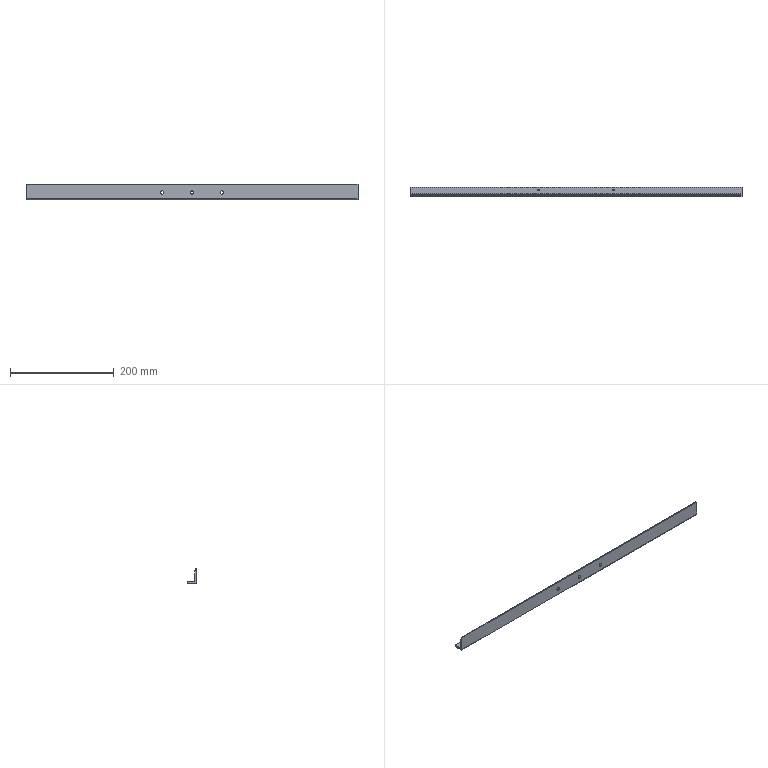Component | SolidWorks | CTM-HVS-52-OA-02-15-1 | 1 solid | 22 faces | box 640 x 18 x 30 mm | volume 105761 mm3 | cylinder 12 | plane 10 | commonest cylinder face diameters 6.6 x6 3.3 x4 4 x2 | material 316L
build123d program:
from build123d import *

# Parameters (mm, degrees)
SKETCH1_W             = 640
SKETCH1_H             = 30
EXTRUDE1_DEPTH        = 2
SKETCH2_W             = 640
SKETCH2_H             = 4
EXTRUDE2_DEPTH        = 14
FILLET1_R             = 2
FILLET2_R             = 2
SKETCH3_R             = 3.3
EXTRUDE3_DEPTH        = 321.657
SKETCH4_W             = 2
SKETCH4_H             = 5
CUT_EXTRUDE1_DEPTH    = 641.376
M4_TAPPED_HOLE1_D     = 3.3
M4_TAPPED_HOLE1_DEPTH = 11.5
M4_TAPPED_HOLE1_TIP   = 0.9914


with BuildPart() as part:
    # Sketch1 → Extrude1 (new, symmetric)
    with BuildSketch(Plane.XY):
        Rectangle(SKETCH1_W, SKETCH1_H)
    extrude(amount=EXTRUDE1_DEPTH, both=True)

    # Sketch2 → Extrude2 (add)
    with BuildSketch(Plane.XY.offset(2)):
        with Locations((0, 13)):
            Rectangle(SKETCH2_W, SKETCH2_H)
    extrude(amount=EXTRUDE2_DEPTH)

    # Fillet1
    fillet1_edges = [part.edges().sort_by_distance(p)[0] for p in [
        (0, 15, -2),
    ]]
    fillet(fillet1_edges, radius=FILLET1_R)

    # Fillet2
    fillet2_edges = [part.edges().sort_by_distance(p)[0] for p in [
        (0, 11, 2),
    ]]
    fillet(fillet2_edges, radius=FILLET2_R)

    # Sketch3 → Extrude3 (cut, through all)
    with BuildSketch(Plane.XY.offset(2)):
        with Locations((-57.5, 1)):
            Circle(SKETCH3_R)
        with Locations((0, 1)):
            Circle(SKETCH3_R)
    extrude3 = extrude(amount=-EXTRUDE3_DEPTH, mode=Mode.SUBTRACT)

    # Mirror1: Extrude3 across plane
    add(extrude3.mirror(Plane(origin=(0, 0, 0), x_dir=(0, 0, 1), z_dir=(1, 0, 0))), mode=Mode.SUBTRACT)

    # Sketch4 → Cut-Extrude1 (cut, through all)
    with BuildSketch(Plane.ZY.offset(320)):
        with Locations((1, -12.5)):
            Rectangle(SKETCH4_W, SKETCH4_H)
    extrude(amount=-CUT_EXTRUDE1_DEPTH, mode=Mode.SUBTRACT)

    # M4 Tapped Hole1
    with Locations(Plane.XZ.offset(-11)):
        with Locations((-72.5, 11), (72.5, 11)):
            Hole(M4_TAPPED_HOLE1_D / 2, depth=M4_TAPPED_HOLE1_DEPTH)
            with Locations((0, 0, -(M4_TAPPED_HOLE1_DEPTH + M4_TAPPED_HOLE1_TIP / 2))):  # 118° drill point
                Cone(0, M4_TAPPED_HOLE1_D / 2, M4_TAPPED_HOLE1_TIP, mode=Mode.SUBTRACT)


solid = part.part

# Placed as in the assembly
solid = solid.moved(Location((-22.307, -58.557, 37.5), (-90, 0, 0)))
STEP:
#1=CARTESIAN_POINT('',(-3.733,-1.807,0.8858));
#2=VERTEX_POINT('',#1);
#3=CARTESIAN_POINT('',(-3.733,-1.937,0.8858));
#4=VERTEX_POINT('',#3);
#5=CARTESIAN_POINT('',(-3.733,-1.872,0.8858));
#6=DIRECTION('',(-0.,-0.,1.));
#7=DIRECTION('',(0.,-1.,0.));
#8=AXIS2_PLACEMENT_3D('',#5,#6,#7);
#9=CIRCLE('',#8,0.06496);
#10=EDGE_CURVE('',#2,#4,#9,.T.);
#11=ORIENTED_EDGE('',*,*,#10,.F.);
#12=CARTESIAN_POINT('',(-3.733,-1.807,1.043));
#13=VERTEX_POINT('',#12);
#14=CARTESIAN_POINT('',(-3.733,-1.807,1.043));
#15=DIRECTION('',(-0.,-0.,1.));
#16=VECTOR('',#15,39.37);
#17=LINE('',#14,#16);
#18=EDGE_CURVE('',#2,#13,#17,.T.);
#19=ORIENTED_EDGE('',*,*,#18,.T.);
#20=CARTESIAN_POINT('',(-3.733,-1.937,1.043));
#21=VERTEX_POINT('',#20);
#22=CARTESIAN_POINT('',(-3.733,-1.872,1.043));
#23=DIRECTION('',(-0.,-0.,1.));
#24=DIRECTION('',(0.,-1.,0.));
#25=AXIS2_PLACEMENT_3D('',#22,#23,#24);
#26=CIRCLE('',#25,0.06496);
#27=EDGE_CURVE('',#13,#21,#26,.T.);
#28=ORIENTED_EDGE('',*,*,#27,.T.);
#29=CARTESIAN_POINT('',(-3.733,-1.937,1.043));
#30=DIRECTION('',(-0.,-0.,1.));
#31=VECTOR('',#30,39.37);
#32=LINE('',#29,#31);
#33=EDGE_CURVE('',#4,#21,#32,.T.);
#34=ORIENTED_EDGE('',*,*,#33,.F.);
#35=EDGE_LOOP('',(#11,#19,#28,#34));
#36=FACE_OUTER_BOUND('',#35,.T.);
#37=CARTESIAN_POINT('',(-3.733,-1.872,1.043));
#38=DIRECTION('',(-0.,-0.,1.));
#39=DIRECTION('',(0.,-1.,0.));
#40=AXIS2_PLACEMENT_3D('',#37,#38,#39);
#41=CYLINDRICAL_SURFACE('',#40,0.06496);
#42=ADVANCED_FACE('',(#36),#41,.F.);
#43=CARTESIAN_POINT('',(1.976,-1.807,0.8858));
#44=VERTEX_POINT('',#43);
#45=CARTESIAN_POINT('',(1.976,-1.937,0.8858));
#46=VERTEX_POINT('',#45);
#47=CARTESIAN_POINT('',(1.976,-1.872,0.8858));
#48=DIRECTION('',(-0.,-0.,1.));
#49=DIRECTION('',(0.,-1.,0.));
#50=AXIS2_PLACEMENT_3D('',#47,#48,#49);
#51=CIRCLE('',#50,0.06496);
#52=EDGE_CURVE('',#44,#46,#51,.T.);
#53=ORIENTED_EDGE('',*,*,#52,.F.);
#54=CARTESIAN_POINT('',(1.976,-1.807,1.043));
#55=VERTEX_POINT('',#54);
#56=CARTESIAN_POINT('',(1.976,-1.807,1.043));
#57=DIRECTION('',(-0.,-0.,1.));
#58=VECTOR('',#57,39.37);
#59=LINE('',#56,#58);
#60=EDGE_CURVE('',#44,#55,#59,.T.);
#61=ORIENTED_EDGE('',*,*,#60,.T.);
#62=CARTESIAN_POINT('',(1.976,-1.937,1.043));
#63=VERTEX_POINT('',#62);
#64=CARTESIAN_POINT('',(1.976,-1.872,1.043));
#65=DIRECTION('',(-0.,-0.,1.));
#66=DIRECTION('',(0.,-1.,0.));
#67=AXIS2_PLACEMENT_3D('',#64,#65,#66);
#68=CIRCLE('',#67,0.06496);
#69=EDGE_CURVE('',#55,#63,#68,.T.);
#70=ORIENTED_EDGE('',*,*,#69,.T.);
#71=CARTESIAN_POINT('',(1.976,-1.937,1.043));
#72=DIRECTION('',(-0.,-0.,1.));
#73=VECTOR('',#72,39.37);
#74=LINE('',#71,#73);
#75=EDGE_CURVE('',#46,#63,#74,.T.);
#76=ORIENTED_EDGE('',*,*,#75,.F.);
#77=EDGE_LOOP('',(#53,#61,#70,#76));
#78=FACE_OUTER_BOUND('',#77,.T.);
#79=CARTESIAN_POINT('',(1.976,-1.872,1.043));
#80=DIRECTION('',(-0.,-0.,1.));
#81=DIRECTION('',(0.,-1.,0.));
#82=AXIS2_PLACEMENT_3D('',#79,#80,#81);
#83=CYLINDRICAL_SURFACE('',#82,0.06496);
#84=ADVANCED_FACE('',(#78),#83,.F.);
#85=CARTESIAN_POINT('',(1.515,-2.384,1.437));
#86=VERTEX_POINT('',#85);
#87=CARTESIAN_POINT('',(1.256,-2.384,1.437));
#88=VERTEX_POINT('',#87);
#89=CARTESIAN_POINT('',(1.386,-2.384,1.437));
#90=DIRECTION('',(-0.,-1.,-0.));
#91=DIRECTION('',(-1.,0.,-0.));
#92=AXIS2_PLACEMENT_3D('',#89,#90,#91);
#93=CIRCLE('',#92,0.1299);
#94=EDGE_CURVE('',#86,#88,#93,.T.);
#95=ORIENTED_EDGE('',*,*,#94,.T.);
#96=CARTESIAN_POINT('',(1.256,-2.227,1.437));
#97=VERTEX_POINT('',#96);
#98=CARTESIAN_POINT('',(1.256,-2.384,1.437));
#99=DIRECTION('',(0.,1.,0.));
#100=VECTOR('',#99,39.37);
#101=LINE('',#98,#100);
#102=EDGE_CURVE('',#88,#97,#101,.T.);
#103=ORIENTED_EDGE('',*,*,#102,.T.);
#104=CARTESIAN_POINT('',(1.515,-2.227,1.437));
#105=VERTEX_POINT('',#104);
#106=CARTESIAN_POINT('',(1.386,-2.227,1.437));
#107=DIRECTION('',(-0.,-1.,-0.));
#108=DIRECTION('',(-1.,0.,-0.));
#109=AXIS2_PLACEMENT_3D('',#106,#107,#108);
#110=CIRCLE('',#109,0.1299);
#111=EDGE_CURVE('',#105,#97,#110,.T.);
#112=ORIENTED_EDGE('',*,*,#111,.F.);
#113=CARTESIAN_POINT('',(1.515,-2.384,1.437));
#114=DIRECTION('',(0.,1.,0.));
#115=VECTOR('',#114,39.37);
#116=LINE('',#113,#115);
#117=EDGE_CURVE('',#86,#105,#116,.T.);
#118=ORIENTED_EDGE('',*,*,#117,.F.);
#119=EDGE_LOOP('',(#95,#103,#112,#118));
#120=FACE_OUTER_BOUND('',#119,.T.);
#121=CARTESIAN_POINT('',(1.386,-2.384,1.437));
#122=DIRECTION('',(0.,1.,0.));
#123=DIRECTION('',(1.,0.,0.));
#124=AXIS2_PLACEMENT_3D('',#121,#122,#123);
#125=CYLINDRICAL_SURFACE('',#124,0.1299);
#126=ADVANCED_FACE('',(#120),#125,.F.);
#127=CARTESIAN_POINT('',(-1.008,-2.384,1.437));
#128=VERTEX_POINT('',#127);
#129=CARTESIAN_POINT('',(-0.7483,-2.384,1.437));
#130=VERTEX_POINT('',#129);
#131=CARTESIAN_POINT('',(-0.8782,-2.384,1.437));
#132=DIRECTION('',(0.,1.,0.));
#133=DIRECTION('',(1.,0.,0.));
#134=AXIS2_PLACEMENT_3D('',#131,#132,#133);
#135=CIRCLE('',#134,0.1299);
#136=EDGE_CURVE('',#128,#130,#135,.T.);
#137=ORIENTED_EDGE('',*,*,#136,.F.);
#138=CARTESIAN_POINT('',(-1.008,-2.227,1.437));
#139=VERTEX_POINT('',#138);
#140=CARTESIAN_POINT('',(-1.008,-2.384,1.437));
#141=DIRECTION('',(0.,1.,0.));
#142=VECTOR('',#141,39.37);
#143=LINE('',#140,#142);
#144=EDGE_CURVE('',#128,#139,#143,.T.);
#145=ORIENTED_EDGE('',*,*,#144,.T.);
#146=CARTESIAN_POINT('',(-0.7483,-2.227,1.437));
#147=VERTEX_POINT('',#146);
#148=CARTESIAN_POINT('',(-0.8782,-2.227,1.437));
#149=DIRECTION('',(0.,1.,0.));
#150=DIRECTION('',(1.,0.,0.));
#151=AXIS2_PLACEMENT_3D('',#148,#149,#150);
#152=CIRCLE('',#151,0.1299);
#153=EDGE_CURVE('',#139,#147,#152,.T.);
#154=ORIENTED_EDGE('',*,*,#153,.T.);
#155=CARTESIAN_POINT('',(-0.7483,-2.384,1.437));
#156=DIRECTION('',(0.,1.,0.));
#157=VECTOR('',#156,39.37);
#158=LINE('',#155,#157);
#159=EDGE_CURVE('',#130,#147,#158,.T.);
#160=ORIENTED_EDGE('',*,*,#159,.F.);
#161=EDGE_LOOP('',(#137,#145,#154,#160));
#162=FACE_OUTER_BOUND('',#161,.T.);
#163=CARTESIAN_POINT('',(-0.8782,-2.384,1.437));
#164=DIRECTION('',(0.,1.,0.));
#165=DIRECTION('',(1.,0.,0.));
#166=AXIS2_PLACEMENT_3D('',#163,#164,#165);
#167=CYLINDRICAL_SURFACE('',#166,0.1299);
#168=ADVANCED_FACE('',(#162),#167,.F.);
#169=CARTESIAN_POINT('',(-3.272,-2.384,1.437));
#170=VERTEX_POINT('',#169);
#171=CARTESIAN_POINT('',(-3.012,-2.384,1.437));
#172=VERTEX_POINT('',#171);
#173=CARTESIAN_POINT('',(-3.142,-2.384,1.437));
#174=DIRECTION('',(0.,1.,0.));
#175=DIRECTION('',(1.,0.,0.));
#176=AXIS2_PLACEMENT_3D('',#173,#174,#175);
#177=CIRCLE('',#176,0.1299);
#178=EDGE_CURVE('',#170,#172,#177,.T.);
#179=ORIENTED_EDGE('',*,*,#178,.F.);
#180=CARTESIAN_POINT('',(-3.272,-2.227,1.437));
#181=VERTEX_POINT('',#180);
#182=CARTESIAN_POINT('',(-3.272,-2.384,1.437));
#183=DIRECTION('',(0.,1.,0.));
#184=VECTOR('',#183,39.37);
#185=LINE('',#182,#184);
#186=EDGE_CURVE('',#170,#181,#185,.T.);
#187=ORIENTED_EDGE('',*,*,#186,.T.);
#188=CARTESIAN_POINT('',(-3.012,-2.227,1.437));
#189=VERTEX_POINT('',#188);
#190=CARTESIAN_POINT('',(-3.142,-2.227,1.437));
#191=DIRECTION('',(0.,1.,0.));
#192=DIRECTION('',(1.,0.,0.));
#193=AXIS2_PLACEMENT_3D('',#190,#191,#192);
#194=CIRCLE('',#193,0.1299);
#195=EDGE_CURVE('',#181,#189,#194,.T.);
#196=ORIENTED_EDGE('',*,*,#195,.T.);
#197=CARTESIAN_POINT('',(-3.012,-2.384,1.437));
#198=DIRECTION('',(0.,1.,0.));
#199=VECTOR('',#198,39.37);
#200=LINE('',#197,#199);
#201=EDGE_CURVE('',#172,#189,#200,.T.);
#202=ORIENTED_EDGE('',*,*,#201,.F.);
#203=EDGE_LOOP('',(#179,#187,#196,#202));
#204=FACE_OUTER_BOUND('',#203,.T.);
#205=CARTESIAN_POINT('',(-3.142,-2.384,1.437));
#206=DIRECTION('',(0.,1.,0.));
#207=DIRECTION('',(1.,0.,0.));
#208=AXIS2_PLACEMENT_3D('',#205,#206,#207);
#209=CYLINDRICAL_SURFACE('',#208,0.1299);
#210=ADVANCED_FACE('',(#204),#209,.F.);
#211=CARTESIAN_POINT('',(-13.477,-1.675,1.043));
#212=VERTEX_POINT('',#211);
#213=CARTESIAN_POINT('',(-13.477,-2.148,1.043));
#214=VERTEX_POINT('',#213);
#215=CARTESIAN_POINT('',(-13.477,-1.675,1.043));
#216=DIRECTION('',(-0.,-1.,-0.));
#217=VECTOR('',#216,39.37);
#218=LINE('',#215,#217);
#219=EDGE_CURVE('',#212,#214,#218,.T.);
#220=ORIENTED_EDGE('',*,*,#219,.T.);
#221=CARTESIAN_POINT('',(11.72,-2.148,1.043));
#222=VERTEX_POINT('',#221);
#223=CARTESIAN_POINT('',(-13.477,-2.148,1.043));
#224=DIRECTION('',(1.,-0.,0.));
#225=VECTOR('',#224,39.37);
#226=LINE('',#223,#225);
#227=EDGE_CURVE('',#214,#222,#226,.T.);
#228=ORIENTED_EDGE('',*,*,#227,.T.);
#229=CARTESIAN_POINT('',(11.72,-1.675,1.043));
#230=VERTEX_POINT('',#229);
#231=CARTESIAN_POINT('',(11.72,-1.675,1.043));
#232=DIRECTION('',(-0.,-1.,-0.));
#233=VECTOR('',#232,39.37);
#234=LINE('',#231,#233);
#235=EDGE_CURVE('',#230,#222,#234,.T.);
#236=ORIENTED_EDGE('',*,*,#235,.F.);
#237=CARTESIAN_POINT('',(-13.477,-1.675,1.043));
#238=DIRECTION('',(1.,-0.,0.));
#239=VECTOR('',#238,39.37);
#240=LINE('',#237,#239);
#241=EDGE_CURVE('',#212,#230,#240,.T.);
#242=ORIENTED_EDGE('',*,*,#241,.F.);
#243=EDGE_LOOP('',(#220,#228,#236,#242));
#244=FACE_OUTER_BOUND('',#243,.T.);
#245=CARTESIAN_POINT('',(1.976,-1.872,1.043));
#246=DIRECTION('',(-0.,-0.,1.));
#247=DIRECTION('',(0.,-1.,0.));
#248=AXIS2_PLACEMENT_3D('',#245,#246,#247);
#249=CIRCLE('',#248,0.06496);
#250=EDGE_CURVE('',#63,#55,#249,.T.);
#251=ORIENTED_EDGE('',*,*,#250,.F.);
#252=ORIENTED_EDGE('',*,*,#69,.F.);
#253=EDGE_LOOP('',(#251,#252));
#254=FACE_BOUND('',#253,.T.);
#255=CARTESIAN_POINT('',(-3.733,-1.872,1.043));
#256=DIRECTION('',(-0.,-0.,1.));
#257=DIRECTION('',(0.,-1.,0.));
#258=AXIS2_PLACEMENT_3D('',#255,#256,#257);
#259=CIRCLE('',#258,0.06496);
#260=EDGE_CURVE('',#21,#13,#259,.T.);
#261=ORIENTED_EDGE('',*,*,#260,.F.);
#262=ORIENTED_EDGE('',*,*,#27,.F.);
#263=EDGE_LOOP('',(#261,#262));
#264=FACE_BOUND('',#263,.T.);
#265=CARTESIAN_POINT('',(-13.477,-1.675,1.043));
#266=DIRECTION('',(0.,0.,-1.));
#267=DIRECTION('',(0.,1.,0.));
#268=AXIS2_PLACEMENT_3D('',#265,#266,#267);
#269=PLANE('',#268);
#270=ADVANCED_FACE('',(#244,#254,#264),#269,.F.);
#271=CARTESIAN_POINT('',(11.72,-2.227,1.87));
#272=VERTEX_POINT('',#271);
#273=CARTESIAN_POINT('',(-13.477,-2.227,1.87));
#274=VERTEX_POINT('',#273);
#275=CARTESIAN_POINT('',(11.72,-2.227,1.87));
#276=DIRECTION('',(-1.,0.,-0.));
#277=VECTOR('',#276,39.37);
#278=LINE('',#275,#277);
#279=EDGE_CURVE('',#272,#274,#278,.T.);
#280=ORIENTED_EDGE('',*,*,#279,.F.);
#281=CARTESIAN_POINT('',(11.72,-2.227,1.122));
#282=VERTEX_POINT('',#281);
#283=CARTESIAN_POINT('',(11.72,-2.227,0.8858));
#284=DIRECTION('',(0.,0.,-1.));
#285=VECTOR('',#284,39.37);
#286=LINE('',#283,#285);
#287=EDGE_CURVE('',#272,#282,#286,.T.);
#288=ORIENTED_EDGE('',*,*,#287,.T.);
#289=CARTESIAN_POINT('',(-13.477,-2.227,1.122));
#290=VERTEX_POINT('',#289);
#291=CARTESIAN_POINT('',(11.72,-2.227,1.122));
#292=DIRECTION('',(-1.,0.,-0.));
#293=VECTOR('',#292,39.37);
#294=LINE('',#291,#293);
#295=EDGE_CURVE('',#282,#290,#294,.T.);
#296=ORIENTED_EDGE('',*,*,#295,.T.);
#297=CARTESIAN_POINT('',(-13.477,-2.227,0.8858));
#298=DIRECTION('',(-0.,-0.,1.));
#299=VECTOR('',#298,39.37);
#300=LINE('',#297,#299);
#301=EDGE_CURVE('',#290,#274,#300,.T.);
#302=ORIENTED_EDGE('',*,*,#301,.T.);
#303=EDGE_LOOP('',(#280,#288,#296,#302));
#304=FACE_OUTER_BOUND('',#303,.T.);
#305=CARTESIAN_POINT('',(-3.142,-2.227,1.437));
#306=DIRECTION('',(0.,1.,0.));
#307=DIRECTION('',(1.,0.,0.));
#308=AXIS2_PLACEMENT_3D('',#305,#306,#307);
#309=CIRCLE('',#308,0.1299);
#310=EDGE_CURVE('',#189,#181,#309,.T.);
#311=ORIENTED_EDGE('',*,*,#310,.F.);
#312=ORIENTED_EDGE('',*,*,#195,.F.);
#313=EDGE_LOOP('',(#311,#312));
#314=FACE_BOUND('',#313,.T.);
#315=CARTESIAN_POINT('',(-0.8782,-2.227,1.437));
#316=DIRECTION('',(0.,1.,0.));
#317=DIRECTION('',(1.,0.,0.));
#318=AXIS2_PLACEMENT_3D('',#315,#316,#317);
#319=CIRCLE('',#318,0.1299);
#320=EDGE_CURVE('',#147,#139,#319,.T.);
#321=ORIENTED_EDGE('',*,*,#320,.F.);
#322=ORIENTED_EDGE('',*,*,#153,.F.);
#323=EDGE_LOOP('',(#321,#322));
#324=FACE_BOUND('',#323,.T.);
#325=ORIENTED_EDGE('',*,*,#111,.T.);
#326=CARTESIAN_POINT('',(1.386,-2.227,1.437));
#327=DIRECTION('',(-0.,-1.,-0.));
#328=DIRECTION('',(-1.,0.,-0.));
#329=AXIS2_PLACEMENT_3D('',#326,#327,#328);
#330=CIRCLE('',#329,0.1299);
#331=EDGE_CURVE('',#97,#105,#330,.T.);
#332=ORIENTED_EDGE('',*,*,#331,.T.);
#333=EDGE_LOOP('',(#325,#332));
#334=FACE_BOUND('',#333,.T.);
#335=CARTESIAN_POINT('',(11.72,-2.227,2.067));
#336=DIRECTION('',(0.,1.,0.));
#337=DIRECTION('',(1.,-0.,0.));
#338=AXIS2_PLACEMENT_3D('',#335,#336,#337);
#339=PLANE('',#338);
#340=ADVANCED_FACE('',(#304,#314,#324,#334),#339,.T.);
#341=CARTESIAN_POINT('',(-13.477,-2.384,0.9646));
#342=VERTEX_POINT('',#341);
#343=CARTESIAN_POINT('',(-13.477,-2.384,2.067));
#344=VERTEX_POINT('',#343);
#345=CARTESIAN_POINT('',(-13.477,-2.384,0.8858));
#346=DIRECTION('',(-0.,-0.,1.));
#347=VECTOR('',#346,39.37);
#348=LINE('',#345,#347);
#349=EDGE_CURVE('',#342,#344,#348,.T.);
#350=ORIENTED_EDGE('',*,*,#349,.F.);
#351=CARTESIAN_POINT('',(11.72,-2.384,0.9646));
#352=VERTEX_POINT('',#351);
#353=CARTESIAN_POINT('',(11.72,-2.384,0.9646));
#354=DIRECTION('',(1.,-0.,0.));
#355=VECTOR('',#354,39.37);
#356=LINE('',#353,#355);
#357=EDGE_CURVE('',#342,#352,#356,.T.);
#358=ORIENTED_EDGE('',*,*,#357,.T.);
#359=CARTESIAN_POINT('',(11.72,-2.384,2.067));
#360=VERTEX_POINT('',#359);
#361=CARTESIAN_POINT('',(11.72,-2.384,0.8858));
#362=DIRECTION('',(0.,0.,-1.));
#363=VECTOR('',#362,39.37);
#364=LINE('',#361,#363);
#365=EDGE_CURVE('',#360,#352,#364,.T.);
#366=ORIENTED_EDGE('',*,*,#365,.F.);
#367=CARTESIAN_POINT('',(-13.477,-2.384,2.067));
#368=DIRECTION('',(1.,-0.,0.));
#369=VECTOR('',#368,39.37);
#370=LINE('',#367,#369);
#371=EDGE_CURVE('',#344,#360,#370,.T.);
#372=ORIENTED_EDGE('',*,*,#371,.F.);
#373=EDGE_LOOP('',(#350,#358,#366,#372));
#374=FACE_OUTER_BOUND('',#373,.T.);
#375=CARTESIAN_POINT('',(-3.142,-2.384,1.437));
#376=DIRECTION('',(0.,1.,0.));
#377=DIRECTION('',(1.,0.,0.));
#378=AXIS2_PLACEMENT_3D('',#375,#376,#377);
#379=CIRCLE('',#378,0.1299);
#380=EDGE_CURVE('',#172,#170,#379,.T.);
#381=ORIENTED_EDGE('',*,*,#380,.T.);
#382=ORIENTED_EDGE('',*,*,#178,.T.);
#383=EDGE_LOOP('',(#381,#382));
#384=FACE_BOUND('',#383,.T.);
#385=CARTESIAN_POINT('',(-0.8782,-2.384,1.437));
#386=DIRECTION('',(0.,1.,0.));
#387=DIRECTION('',(1.,0.,0.));
#388=AXIS2_PLACEMENT_3D('',#385,#386,#387);
#389=CIRCLE('',#388,0.1299);
#390=EDGE_CURVE('',#130,#128,#389,.T.);
#391=ORIENTED_EDGE('',*,*,#390,.T.);
#392=ORIENTED_EDGE('',*,*,#136,.T.);
#393=EDGE_LOOP('',(#391,#392));
#394=FACE_BOUND('',#393,.T.);
#395=ORIENTED_EDGE('',*,*,#94,.F.);
#396=CARTESIAN_POINT('',(1.386,-2.384,1.437));
#397=DIRECTION('',(-0.,-1.,-0.));
#398=DIRECTION('',(-1.,0.,-0.));
#399=AXIS2_PLACEMENT_3D('',#396,#397,#398);
#400=CIRCLE('',#399,0.1299);
#401=EDGE_CURVE('',#88,#86,#400,.T.);
#402=ORIENTED_EDGE('',*,*,#401,.F.);
#403=EDGE_LOOP('',(#395,#402));
#404=FACE_BOUND('',#403,.T.);
#405=CARTESIAN_POINT('',(11.72,-2.384,2.067));
#406=DIRECTION('',(0.,1.,0.));
#407=DIRECTION('',(1.,-0.,0.));
#408=AXIS2_PLACEMENT_3D('',#405,#406,#407);
#409=PLANE('',#408);
#410=ADVANCED_FACE('',(#374,#384,#394,#404),#409,.F.);
#411=CARTESIAN_POINT('',(11.72,-2.305,1.87));
#412=VERTEX_POINT('',#411);
#413=CARTESIAN_POINT('',(11.72,-2.227,1.87));
#414=DIRECTION('',(-0.,-1.,-0.));
#415=VECTOR('',#414,39.37);
#416=LINE('',#413,#415);
#417=EDGE_CURVE('',#272,#412,#416,.T.);
#418=ORIENTED_EDGE('',*,*,#417,.T.);
#419=CARTESIAN_POINT('',(11.72,-2.305,2.067));
#420=VERTEX_POINT('',#419);
#421=CARTESIAN_POINT('',(11.72,-2.305,2.067));
#422=DIRECTION('',(-0.,-0.,1.));
#423=VECTOR('',#422,39.37);
#424=LINE('',#421,#423);
#425=EDGE_CURVE('',#412,#420,#424,.T.);
#426=ORIENTED_EDGE('',*,*,#425,.T.);
#427=CARTESIAN_POINT('',(11.72,-2.227,2.067));
#428=DIRECTION('',(-0.,-1.,-0.));
#429=VECTOR('',#428,39.37);
#430=LINE('',#427,#429);
#431=EDGE_CURVE('',#420,#360,#430,.T.);
#432=ORIENTED_EDGE('',*,*,#431,.T.);
#433=ORIENTED_EDGE('',*,*,#365,.T.);
#434=CARTESIAN_POINT('',(11.72,-2.305,0.8858));
#435=VERTEX_POINT('',#434);
#436=CARTESIAN_POINT('',(11.72,-2.305,0.9646));
#437=DIRECTION('',(1.,-0.,0.));
#438=DIRECTION('',(0.,1.,0.));
#439=AXIS2_PLACEMENT_3D('',#436,#437,#438);
#440=CIRCLE('',#439,0.07874);
#441=EDGE_CURVE('',#352,#435,#440,.T.);
#442=ORIENTED_EDGE('',*,*,#441,.T.);
#443=CARTESIAN_POINT('',(11.72,-1.675,0.8858));
#444=VERTEX_POINT('',#443);
#445=CARTESIAN_POINT('',(11.72,-2.227,0.8858));
#446=DIRECTION('',(-0.,-1.,-0.));
#447=VECTOR('',#446,39.37);
#448=LINE('',#445,#447);
#449=EDGE_CURVE('',#444,#435,#448,.T.);
#450=ORIENTED_EDGE('',*,*,#449,.F.);
#451=CARTESIAN_POINT('',(11.72,-1.675,1.043));
#452=DIRECTION('',(0.,0.,-1.));
#453=VECTOR('',#452,39.37);
#454=LINE('',#451,#453);
#455=EDGE_CURVE('',#230,#444,#454,.T.);
#456=ORIENTED_EDGE('',*,*,#455,.F.);
#457=ORIENTED_EDGE('',*,*,#235,.T.);
#458=CARTESIAN_POINT('',(11.72,-2.148,1.122));
#459=DIRECTION('',(-1.,0.,-0.));
#460=DIRECTION('',(0.,1.,0.));
#461=AXIS2_PLACEMENT_3D('',#458,#459,#460);
#462=CIRCLE('',#461,0.07874);
#463=EDGE_CURVE('',#222,#282,#462,.T.);
#464=ORIENTED_EDGE('',*,*,#463,.T.);
#465=ORIENTED_EDGE('',*,*,#287,.F.);
#466=EDGE_LOOP('',(#418,#426,#432,#433,#442,#450,#456,#457,#464,#465));
#467=FACE_OUTER_BOUND('',#466,.T.);
#468=CARTESIAN_POINT('',(11.72,-2.227,0.8858));
#469=DIRECTION('',(-1.,0.,-0.));
#470=DIRECTION('',(0.,1.,0.));
#471=AXIS2_PLACEMENT_3D('',#468,#469,#470);
#472=PLANE('',#471);
#473=ADVANCED_FACE('',(#467),#472,.F.);
#474=CARTESIAN_POINT('',(-3.733,-1.872,0.8858));
#475=DIRECTION('',(-0.,-0.,1.));
#476=DIRECTION('',(0.,-1.,0.));
#477=AXIS2_PLACEMENT_3D('',#474,#475,#476);
#478=CIRCLE('',#477,0.06496);
#479=EDGE_CURVE('',#4,#2,#478,.T.);
#480=ORIENTED_EDGE('',*,*,#479,.T.);
#481=ORIENTED_EDGE('',*,*,#10,.T.);
#482=EDGE_LOOP('',(#480,#481));
#483=FACE_BOUND('',#482,.T.);
#484=CARTESIAN_POINT('',(1.976,-1.872,0.8858));
#485=DIRECTION('',(-0.,-0.,1.));
#486=DIRECTION('',(0.,-1.,0.));
#487=AXIS2_PLACEMENT_3D('',#484,#485,#486);
#488=CIRCLE('',#487,0.06496);
#489=EDGE_CURVE('',#46,#44,#488,.T.);
#490=ORIENTED_EDGE('',*,*,#489,.T.);
#491=ORIENTED_EDGE('',*,*,#52,.T.);
#492=EDGE_LOOP('',(#490,#491));
#493=FACE_BOUND('',#492,.T.);
#494=ORIENTED_EDGE('',*,*,#449,.T.);
#495=CARTESIAN_POINT('',(-13.477,-2.305,0.8858));
#496=VERTEX_POINT('',#495);
#497=CARTESIAN_POINT('',(-13.477,-2.305,0.8858));
#498=DIRECTION('',(-1.,0.,-0.));
#499=VECTOR('',#498,39.37);
#500=LINE('',#497,#499);
#501=EDGE_CURVE('',#435,#496,#500,.T.);
#502=ORIENTED_EDGE('',*,*,#501,.T.);
#503=CARTESIAN_POINT('',(-13.477,-1.675,0.8858));
#504=VERTEX_POINT('',#503);
#505=CARTESIAN_POINT('',(-13.477,-2.227,0.8858));
#506=DIRECTION('',(-0.,-1.,-0.));
#507=VECTOR('',#506,39.37);
#508=LINE('',#505,#507);
#509=EDGE_CURVE('',#504,#496,#508,.T.);
#510=ORIENTED_EDGE('',*,*,#509,.F.);
#511=CARTESIAN_POINT('',(-13.477,-1.675,0.8858));
#512=DIRECTION('',(-1.,0.,-0.));
#513=VECTOR('',#512,39.37);
#514=LINE('',#511,#513);
#515=EDGE_CURVE('',#444,#504,#514,.T.);
#516=ORIENTED_EDGE('',*,*,#515,.F.);
#517=EDGE_LOOP('',(#494,#502,#510,#516));
#518=FACE_OUTER_BOUND('',#517,.T.);
#519=CARTESIAN_POINT('',(-13.477,-2.227,0.8858));
#520=DIRECTION('',(-0.,-0.,1.));
#521=DIRECTION('',(-0.,-1.,-0.));
#522=AXIS2_PLACEMENT_3D('',#519,#520,#521);
#523=PLANE('',#522);
#524=ADVANCED_FACE('',(#483,#493,#518),#523,.F.);
#525=CARTESIAN_POINT('',(-13.477,-2.305,2.067));
#526=VERTEX_POINT('',#525);
#527=CARTESIAN_POINT('',(-13.477,-2.227,2.067));
#528=DIRECTION('',(-0.,-1.,-0.));
#529=VECTOR('',#528,39.37);
#530=LINE('',#527,#529);
#531=EDGE_CURVE('',#526,#344,#530,.T.);
#532=ORIENTED_EDGE('',*,*,#531,.F.);
#533=CARTESIAN_POINT('',(-13.477,-2.305,1.87));
#534=VERTEX_POINT('',#533);
#535=CARTESIAN_POINT('',(-13.477,-2.305,2.067));
#536=DIRECTION('',(-0.,-0.,1.));
#537=VECTOR('',#536,39.37);
#538=LINE('',#535,#537);
#539=EDGE_CURVE('',#534,#526,#538,.T.);
#540=ORIENTED_EDGE('',*,*,#539,.F.);
#541=CARTESIAN_POINT('',(-13.477,-2.227,1.87));
#542=DIRECTION('',(-0.,-1.,-0.));
#543=VECTOR('',#542,39.37);
#544=LINE('',#541,#543);
#545=EDGE_CURVE('',#274,#534,#544,.T.);
#546=ORIENTED_EDGE('',*,*,#545,.F.);
#547=ORIENTED_EDGE('',*,*,#301,.F.);
#548=CARTESIAN_POINT('',(-13.477,-2.148,1.122));
#549=DIRECTION('',(1.,-0.,0.));
#550=DIRECTION('',(0.,-1.,0.));
#551=AXIS2_PLACEMENT_3D('',#548,#549,#550);
#552=CIRCLE('',#551,0.07874);
#553=EDGE_CURVE('',#290,#214,#552,.T.);
#554=ORIENTED_EDGE('',*,*,#553,.T.);
#555=ORIENTED_EDGE('',*,*,#219,.F.);
#556=CARTESIAN_POINT('',(-13.477,-1.675,1.043));
#557=DIRECTION('',(-0.,-0.,1.));
#558=VECTOR('',#557,39.37);
#559=LINE('',#556,#558);
#560=EDGE_CURVE('',#504,#212,#559,.T.);
#561=ORIENTED_EDGE('',*,*,#560,.F.);
#562=ORIENTED_EDGE('',*,*,#509,.T.);
#563=CARTESIAN_POINT('',(-13.477,-2.305,0.9646));
#564=DIRECTION('',(-1.,0.,-0.));
#565=DIRECTION('',(0.,-1.,0.));
#566=AXIS2_PLACEMENT_3D('',#563,#564,#565);
#567=CIRCLE('',#566,0.07874);
#568=EDGE_CURVE('',#496,#342,#567,.T.);
#569=ORIENTED_EDGE('',*,*,#568,.T.);
#570=ORIENTED_EDGE('',*,*,#349,.T.);
#571=EDGE_LOOP('',(#532,#540,#546,#547,#554,#555,#561,#562,#569,#570));
#572=FACE_OUTER_BOUND('',#571,.T.);
#573=CARTESIAN_POINT('',(-13.477,-2.227,0.8858));
#574=DIRECTION('',(1.,-0.,0.));
#575=DIRECTION('',(-0.,-1.,-0.));
#576=AXIS2_PLACEMENT_3D('',#573,#574,#575);
#577=PLANE('',#576);
#578=ADVANCED_FACE('',(#572),#577,.F.);
#579=ORIENTED_EDGE('',*,*,#431,.F.);
#580=CARTESIAN_POINT('',(11.72,-2.305,2.067));
#581=DIRECTION('',(-1.,0.,-0.));
#582=VECTOR('',#581,39.37);
#583=LINE('',#580,#582);
#584=EDGE_CURVE('',#420,#526,#583,.T.);
#585=ORIENTED_EDGE('',*,*,#584,.T.);
#586=ORIENTED_EDGE('',*,*,#531,.T.);
#587=ORIENTED_EDGE('',*,*,#371,.T.);
#588=EDGE_LOOP('',(#579,#585,#586,#587));
#589=FACE_OUTER_BOUND('',#588,.T.);
#590=CARTESIAN_POINT('',(-13.477,-2.227,2.067));
#591=DIRECTION('',(0.,0.,-1.));
#592=DIRECTION('',(0.,1.,0.));
#593=AXIS2_PLACEMENT_3D('',#590,#591,#592);
#594=PLANE('',#593);
#595=ADVANCED_FACE('',(#589),#594,.F.);
#596=ORIENTED_EDGE('',*,*,#455,.T.);
#597=ORIENTED_EDGE('',*,*,#515,.T.);
#598=ORIENTED_EDGE('',*,*,#560,.T.);
#599=ORIENTED_EDGE('',*,*,#241,.T.);
#600=EDGE_LOOP('',(#596,#597,#598,#599));
#601=FACE_OUTER_BOUND('',#600,.T.);
#602=CARTESIAN_POINT('',(11.72,-1.675,0.8858));
#603=DIRECTION('',(-0.,-1.,-0.));
#604=DIRECTION('',(-1.,0.,-0.));
#605=AXIS2_PLACEMENT_3D('',#602,#603,#604);
#606=PLANE('',#605);
#607=ADVANCED_FACE('',(#601),#606,.F.);
#608=ORIENTED_EDGE('',*,*,#441,.F.);
#609=ORIENTED_EDGE('',*,*,#357,.F.);
#610=ORIENTED_EDGE('',*,*,#568,.F.);
#611=ORIENTED_EDGE('',*,*,#501,.F.);
#612=EDGE_LOOP('',(#608,#609,#610,#611));
#613=FACE_OUTER_BOUND('',#612,.T.);
#614=CARTESIAN_POINT('',(-13.477,-2.305,0.9646));
#615=DIRECTION('',(-1.,0.,-0.));
#616=DIRECTION('',(0.,1.,0.));
#617=AXIS2_PLACEMENT_3D('',#614,#615,#616);
#618=CYLINDRICAL_SURFACE('',#617,0.07874);
#619=ADVANCED_FACE('',(#613),#618,.T.);
#620=ORIENTED_EDGE('',*,*,#553,.F.);
#621=ORIENTED_EDGE('',*,*,#295,.F.);
#622=ORIENTED_EDGE('',*,*,#463,.F.);
#623=ORIENTED_EDGE('',*,*,#227,.F.);
#624=EDGE_LOOP('',(#620,#621,#622,#623));
#625=FACE_OUTER_BOUND('',#624,.T.);
#626=CARTESIAN_POINT('',(-13.477,-2.148,1.122));
#627=DIRECTION('',(1.,-0.,0.));
#628=DIRECTION('',(0.,-1.,0.));
#629=AXIS2_PLACEMENT_3D('',#626,#627,#628);
#630=CYLINDRICAL_SURFACE('',#629,0.07874);
#631=ADVANCED_FACE('',(#625),#630,.F.);
#632=ORIENTED_EDGE('',*,*,#186,.F.);
#633=ORIENTED_EDGE('',*,*,#380,.F.);
#634=ORIENTED_EDGE('',*,*,#201,.T.);
#635=ORIENTED_EDGE('',*,*,#310,.T.);
#636=EDGE_LOOP('',(#632,#633,#634,#635));
#637=FACE_OUTER_BOUND('',#636,.T.);
#638=CARTESIAN_POINT('',(-3.142,-2.384,1.437));
#639=DIRECTION('',(0.,1.,0.));
#640=DIRECTION('',(1.,0.,0.));
#641=AXIS2_PLACEMENT_3D('',#638,#639,#640);
#642=CYLINDRICAL_SURFACE('',#641,0.1299);
#643=ADVANCED_FACE('',(#637),#642,.F.);
#644=ORIENTED_EDGE('',*,*,#144,.F.);
#645=ORIENTED_EDGE('',*,*,#390,.F.);
#646=ORIENTED_EDGE('',*,*,#159,.T.);
#647=ORIENTED_EDGE('',*,*,#320,.T.);
#648=EDGE_LOOP('',(#644,#645,#646,#647));
#649=FACE_OUTER_BOUND('',#648,.T.);
#650=CARTESIAN_POINT('',(-0.8782,-2.384,1.437));
#651=DIRECTION('',(0.,1.,0.));
#652=DIRECTION('',(1.,0.,0.));
#653=AXIS2_PLACEMENT_3D('',#650,#651,#652);
#654=CYLINDRICAL_SURFACE('',#653,0.1299);
#655=ADVANCED_FACE('',(#649),#654,.F.);
#656=ORIENTED_EDGE('',*,*,#102,.F.);
#657=ORIENTED_EDGE('',*,*,#401,.T.);
#658=ORIENTED_EDGE('',*,*,#117,.T.);
#659=ORIENTED_EDGE('',*,*,#331,.F.);
#660=EDGE_LOOP('',(#656,#657,#658,#659));
#661=FACE_OUTER_BOUND('',#660,.T.);
#662=CARTESIAN_POINT('',(1.386,-2.384,1.437));
#663=DIRECTION('',(0.,1.,0.));
#664=DIRECTION('',(1.,0.,0.));
#665=AXIS2_PLACEMENT_3D('',#662,#663,#664);
#666=CYLINDRICAL_SURFACE('',#665,0.1299);
#667=ADVANCED_FACE('',(#661),#666,.F.);
#668=ORIENTED_EDGE('',*,*,#539,.T.);
#669=ORIENTED_EDGE('',*,*,#584,.F.);
#670=ORIENTED_EDGE('',*,*,#425,.F.);
#671=CARTESIAN_POINT('',(11.72,-2.305,1.87));
#672=DIRECTION('',(-1.,0.,-0.));
#673=VECTOR('',#672,39.37);
#674=LINE('',#671,#673);
#675=EDGE_CURVE('',#412,#534,#674,.T.);
#676=ORIENTED_EDGE('',*,*,#675,.T.);
#677=EDGE_LOOP('',(#668,#669,#670,#676));
#678=FACE_OUTER_BOUND('',#677,.T.);
#679=CARTESIAN_POINT('',(11.72,-2.305,2.067));
#680=DIRECTION('',(-0.,-1.,-0.));
#681=DIRECTION('',(-1.,0.,-0.));
#682=AXIS2_PLACEMENT_3D('',#679,#680,#681);
#683=PLANE('',#682);
#684=ADVANCED_FACE('',(#678),#683,.F.);
#685=ORIENTED_EDGE('',*,*,#545,.T.);
#686=ORIENTED_EDGE('',*,*,#675,.F.);
#687=ORIENTED_EDGE('',*,*,#417,.F.);
#688=ORIENTED_EDGE('',*,*,#279,.T.);
#689=EDGE_LOOP('',(#685,#686,#687,#688));
#690=FACE_OUTER_BOUND('',#689,.T.);
#691=CARTESIAN_POINT('',(11.72,-2.227,1.87));
#692=DIRECTION('',(0.,0.,-1.));
#693=DIRECTION('',(0.,1.,0.));
#694=AXIS2_PLACEMENT_3D('',#691,#692,#693);
#695=PLANE('',#694);
#696=ADVANCED_FACE('',(#690),#695,.F.);
#697=ORIENTED_EDGE('',*,*,#60,.F.);
#698=ORIENTED_EDGE('',*,*,#489,.F.);
#699=ORIENTED_EDGE('',*,*,#75,.T.);
#700=ORIENTED_EDGE('',*,*,#250,.T.);
#701=EDGE_LOOP('',(#697,#698,#699,#700));
#702=FACE_OUTER_BOUND('',#701,.T.);
#703=CARTESIAN_POINT('',(1.976,-1.872,1.043));
#704=DIRECTION('',(-0.,-0.,1.));
#705=DIRECTION('',(0.,-1.,0.));
#706=AXIS2_PLACEMENT_3D('',#703,#704,#705);
#707=CYLINDRICAL_SURFACE('',#706,0.06496);
#708=ADVANCED_FACE('',(#702),#707,.F.);
#709=ORIENTED_EDGE('',*,*,#18,.F.);
#710=ORIENTED_EDGE('',*,*,#479,.F.);
#711=ORIENTED_EDGE('',*,*,#33,.T.);
#712=ORIENTED_EDGE('',*,*,#260,.T.);
#713=EDGE_LOOP('',(#709,#710,#711,#712));
#714=FACE_OUTER_BOUND('',#713,.T.);
#715=CARTESIAN_POINT('',(-3.733,-1.872,1.043));
#716=DIRECTION('',(-0.,-0.,1.));
#717=DIRECTION('',(0.,-1.,0.));
#718=AXIS2_PLACEMENT_3D('',#715,#716,#717);
#719=CYLINDRICAL_SURFACE('',#718,0.06496);
#720=ADVANCED_FACE('',(#714),#719,.F.);
#721=CLOSED_SHELL('',(#42,#84,#126,#168,#210,#270,#340,#410,#473,#524,#578,#595,#607,#619,#631,#643,#655,#667,#684,#696,#708,#720));
#722=MANIFOLD_SOLID_BREP('',#721);
#723=CARTESIAN_POINT('',(0.,0.,0.));
#724=DIRECTION('',(0.,0.,1.));
#725=DIRECTION('',(1.,0.,0.));
#726=AXIS2_PLACEMENT_3D('',#723,#724,#725);
#727=(LENGTH_UNIT()NAMED_UNIT(*)SI_UNIT($,.METRE.));
#728=LENGTH_MEASURE_WITH_UNIT(LENGTH_MEASURE(0.0254),#727);
#729=DIMENSIONAL_EXPONENTS(1.,0.,0.,0.,0.,0.,0.);
#730=(CONVERSION_BASED_UNIT('',#728)LENGTH_UNIT()NAMED_UNIT(#729));
#731=UNCERTAINTY_MEASURE_WITH_UNIT(LENGTH_MEASURE(0.00001),#730,'','');
#732=(NAMED_UNIT(*)PLANE_ANGLE_UNIT()SI_UNIT($,.RADIAN.));
#733=(NAMED_UNIT(*)SI_UNIT($,.STERADIAN.)SOLID_ANGLE_UNIT());
#734=(GEOMETRIC_REPRESENTATION_CONTEXT(3)GLOBAL_UNCERTAINTY_ASSIGNED_CONTEXT((#731))GLOBAL_UNIT_ASSIGNED_CONTEXT((#730,#732,#733))REPRESENTATION_CONTEXT('',''));
#735=ADVANCED_BREP_SHAPE_REPRESENTATION('',(#722,#726),#734);
#736=COLOUR_RGB('',0.7922,0.8196,0.9333);
#737=FILL_AREA_STYLE_COLOUR('',#736);
#738=FILL_AREA_STYLE('',(#737));
#739=SURFACE_STYLE_FILL_AREA(#738);
#740=SURFACE_SIDE_STYLE('',(#739));
#741=SURFACE_STYLE_USAGE(.BOTH.,#740);
#742=PRESENTATION_STYLE_ASSIGNMENT((#741));
#743=STYLED_ITEM('',(#742),#722);
#744=(LENGTH_UNIT()NAMED_UNIT(*)SI_UNIT($,.METRE.));
#745=LENGTH_MEASURE_WITH_UNIT(LENGTH_MEASURE(0.0254),#744);
#746=DIMENSIONAL_EXPONENTS(1.,0.,0.,0.,0.,0.,0.);
#747=(CONVERSION_BASED_UNIT('',#745)LENGTH_UNIT()NAMED_UNIT(#746));
#748=UNCERTAINTY_MEASURE_WITH_UNIT(LENGTH_MEASURE(0.00001),#747,'','');
#749=(NAMED_UNIT(*)PLANE_ANGLE_UNIT()SI_UNIT($,.RADIAN.));
#750=(NAMED_UNIT(*)SI_UNIT($,.STERADIAN.)SOLID_ANGLE_UNIT());
#751=(GEOMETRIC_REPRESENTATION_CONTEXT(3)GLOBAL_UNCERTAINTY_ASSIGNED_CONTEXT((#748))GLOBAL_UNIT_ASSIGNED_CONTEXT((#747,#749,#750))REPRESENTATION_CONTEXT('',''));
#752=MECHANICAL_DESIGN_GEOMETRIC_PRESENTATION_REPRESENTATION('',(#743),#751);
#753=PRESENTATION_LAYER_ASSIGNMENT('','',(#743));